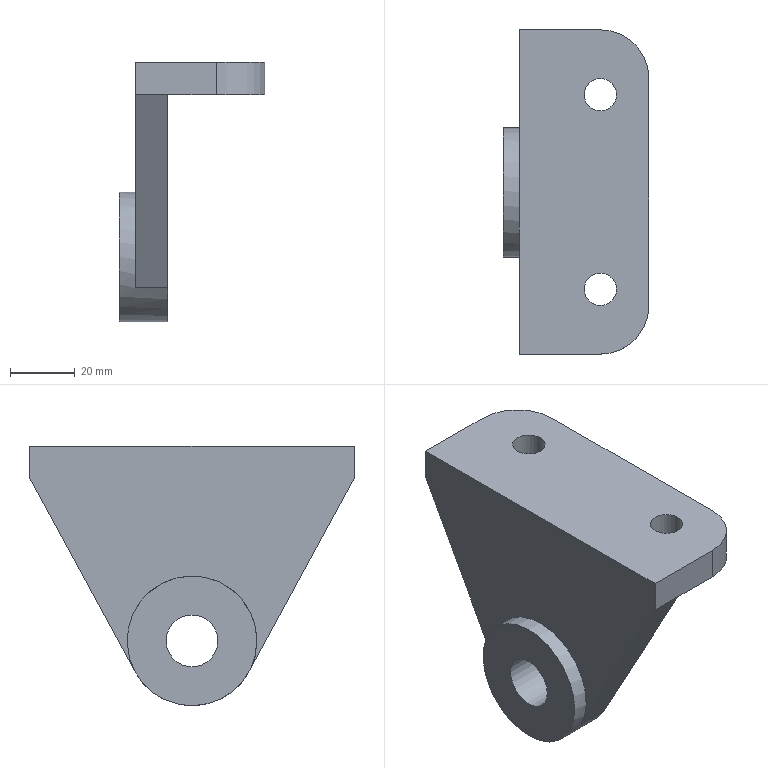Component | NX | SUPORTE_RODA | 1 solid | 16 faces | volume 83584 mm3 | plane 10 | cylinder 6 | commonest cylinder face diameters 30 x2 10 x2 40 x1 16 x1